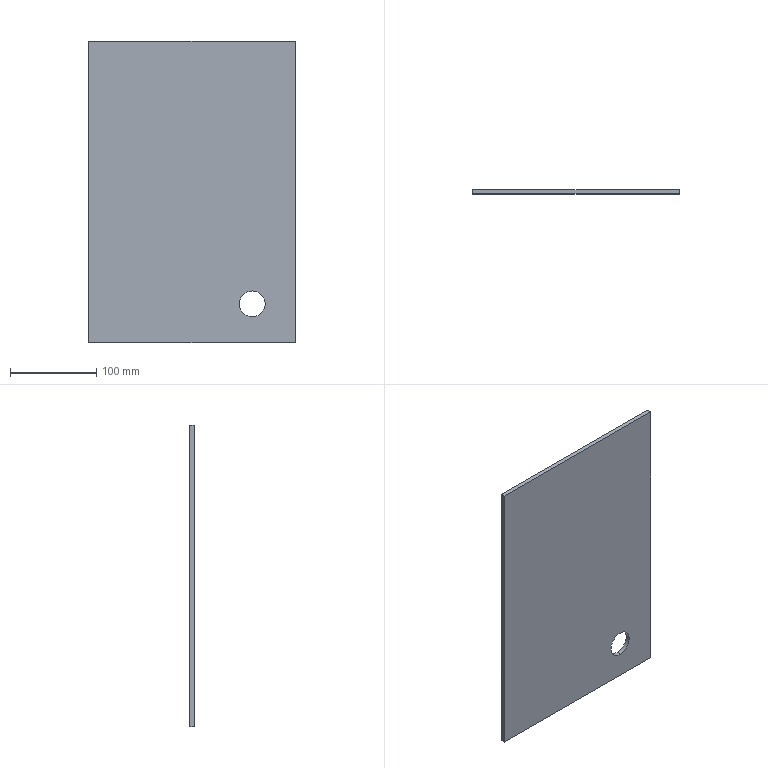Component | SolidWorks | 002FrameBaseAssembly-1_002FrameBasePanel-1 | 1 solid | 8 faces | box 240 x 5 x 350 mm | volume 416466 mm3 | plane 6 | cylinder 2 | commonest cylinder face diameters 30 x2 | material Plain Carbon Steel
build123d program:
from build123d import *

# Parameters (mm, degrees)
SKETCH1_2_W               = 400
SKETCH1_2_H               = 240
BOSS_EXTRUDE1_DEPTH       = 5
CUT_EXTRUDE2_REACH        = 235.292
SKETCH3_R                 = 15
RELIEF_GB6_WEB_DEPTH      = 234.292
RELIEF_GB6_WEB_DEPTH_BACK = 234.292
SKETCH1_W                 = 65
SKETCH1_H                 = 270


with BuildPart() as part:
    # Sketch1_2 → Boss-Extrude1 (new body)
    with BuildSketch(Plane.XY):
        Rectangle(SKETCH1_2_W, SKETCH1_2_H)
    extrude(amount=BOSS_EXTRUDE1_DEPTH)

    # Sketch3 → Cut-Extrude2 (cut, up to next)
    with BuildSketch(Plane.XY.offset(5), mode=Mode.PRIVATE) as cut_extrude2_sk1:
        with Locations((155, 70)):
            Circle(SKETCH3_R)
    cut_extrude2_tool1 = extrude(cut_extrude2_sk1.sketch, amount=-CUT_EXTRUDE2_REACH, mode=Mode.PRIVATE) & part.part
    add(cut_extrude2_tool1.solids().sort_by_distance((155, 70, 5))[0], mode=Mode.SUBTRACT)

    # Sketch1 → Relief_gb6_web (cut, two sides: drawn at the far end of the back side and taken through both)
    with BuildSketch(Plane.XY.offset(-RELIEF_GB6_WEB_DEPTH_BACK)):
        with Locations((-182.5, 0)):
            Rectangle(SKETCH1_W, SKETCH1_H)
    extrude(amount=RELIEF_GB6_WEB_DEPTH + RELIEF_GB6_WEB_DEPTH_BACK, mode=Mode.SUBTRACT)


solid = part.part

# Placed as in the assembly
solid = solid.moved(Location((0, 37, -315), (90, 0, -90)))
STEP:
#1=CARTESIAN_POINT('',(2.756,1.457,-19.094));
#2=VERTEX_POINT('',#1);
#3=CARTESIAN_POINT('',(2.756,1.457,-17.913));
#4=VERTEX_POINT('',#3);
#5=CARTESIAN_POINT('',(2.756,1.457,-18.504));
#6=DIRECTION('',(0.,1.,-0.));
#7=DIRECTION('',(0.,0.,-1.));
#8=AXIS2_PLACEMENT_3D('',#5,#6,#7);
#9=CIRCLE('',#8,0.5906);
#10=EDGE_CURVE('',#2,#4,#9,.T.);
#11=ORIENTED_EDGE('',*,*,#10,.T.);
#12=CARTESIAN_POINT('',(2.756,1.26,-17.913));
#13=VERTEX_POINT('',#12);
#14=CARTESIAN_POINT('',(2.756,1.457,-17.913));
#15=DIRECTION('',(-0.,-1.,0.));
#16=VECTOR('',#15,39.37);
#17=LINE('',#14,#16);
#18=EDGE_CURVE('',#4,#13,#17,.T.);
#19=ORIENTED_EDGE('',*,*,#18,.T.);
#20=CARTESIAN_POINT('',(2.756,1.26,-19.094));
#21=VERTEX_POINT('',#20);
#22=CARTESIAN_POINT('',(2.756,1.26,-18.504));
#23=DIRECTION('',(-0.,-1.,0.));
#24=DIRECTION('',(0.,0.,-1.));
#25=AXIS2_PLACEMENT_3D('',#22,#23,#24);
#26=CIRCLE('',#25,0.5906);
#27=EDGE_CURVE('',#13,#21,#26,.T.);
#28=ORIENTED_EDGE('',*,*,#27,.T.);
#29=CARTESIAN_POINT('',(2.756,1.457,-19.094));
#30=DIRECTION('',(-0.,-1.,0.));
#31=VECTOR('',#30,39.37);
#32=LINE('',#29,#31);
#33=EDGE_CURVE('',#2,#21,#32,.T.);
#34=ORIENTED_EDGE('',*,*,#33,.F.);
#35=EDGE_LOOP('',(#11,#19,#28,#34));
#36=FACE_OUTER_BOUND('',#35,.T.);
#37=CARTESIAN_POINT('',(2.756,1.457,-18.504));
#38=DIRECTION('',(-0.,-1.,0.));
#39=DIRECTION('',(0.,0.,-1.));
#40=AXIS2_PLACEMENT_3D('',#37,#38,#39);
#41=CYLINDRICAL_SURFACE('',#40,0.5906);
#42=ADVANCED_FACE('',(#36),#41,.F.);
#43=CARTESIAN_POINT('',(-4.724,1.457,-20.276));
#44=VERTEX_POINT('',#43);
#45=CARTESIAN_POINT('',(4.724,1.457,-20.276));
#46=VERTEX_POINT('',#45);
#47=CARTESIAN_POINT('',(4.724,1.457,-20.276));
#48=DIRECTION('',(1.,-0.,0.));
#49=VECTOR('',#48,39.37);
#50=LINE('',#47,#49);
#51=EDGE_CURVE('',#44,#46,#50,.T.);
#52=ORIENTED_EDGE('',*,*,#51,.T.);
#53=CARTESIAN_POINT('',(4.724,1.26,-20.276));
#54=VERTEX_POINT('',#53);
#55=CARTESIAN_POINT('',(4.724,1.26,-20.276));
#56=DIRECTION('',(0.,1.,-0.));
#57=VECTOR('',#56,39.37);
#58=LINE('',#55,#57);
#59=EDGE_CURVE('',#54,#46,#58,.T.);
#60=ORIENTED_EDGE('',*,*,#59,.F.);
#61=CARTESIAN_POINT('',(-4.724,1.26,-20.276));
#62=VERTEX_POINT('',#61);
#63=CARTESIAN_POINT('',(4.724,1.26,-20.276));
#64=DIRECTION('',(1.,-0.,0.));
#65=VECTOR('',#64,39.37);
#66=LINE('',#63,#65);
#67=EDGE_CURVE('',#62,#54,#66,.T.);
#68=ORIENTED_EDGE('',*,*,#67,.F.);
#69=CARTESIAN_POINT('',(-4.724,1.26,-20.276));
#70=DIRECTION('',(0.,1.,-0.));
#71=VECTOR('',#70,39.37);
#72=LINE('',#69,#71);
#73=EDGE_CURVE('',#62,#44,#72,.T.);
#74=ORIENTED_EDGE('',*,*,#73,.T.);
#75=EDGE_LOOP('',(#52,#60,#68,#74));
#76=FACE_OUTER_BOUND('',#75,.T.);
#77=CARTESIAN_POINT('',(4.724,1.26,-20.276));
#78=DIRECTION('',(0.,0.,1.));
#79=DIRECTION('',(-0.,-1.,0.));
#80=AXIS2_PLACEMENT_3D('',#77,#78,#79);
#81=PLANE('',#80);
#82=ADVANCED_FACE('',(#76),#81,.F.);
#83=CARTESIAN_POINT('',(4.724,1.457,-6.496));
#84=VERTEX_POINT('',#83);
#85=CARTESIAN_POINT('',(4.724,1.457,-4.528));
#86=DIRECTION('',(0.,0.,1.));
#87=VECTOR('',#86,39.37);
#88=LINE('',#85,#87);
#89=EDGE_CURVE('',#46,#84,#88,.T.);
#90=ORIENTED_EDGE('',*,*,#89,.T.);
#91=CARTESIAN_POINT('',(4.724,1.26,-6.496));
#92=VERTEX_POINT('',#91);
#93=CARTESIAN_POINT('',(4.724,1.26,-6.496));
#94=DIRECTION('',(-0.,-1.,0.));
#95=VECTOR('',#94,39.37);
#96=LINE('',#93,#95);
#97=EDGE_CURVE('',#84,#92,#96,.T.);
#98=ORIENTED_EDGE('',*,*,#97,.T.);
#99=CARTESIAN_POINT('',(4.724,1.26,-4.528));
#100=DIRECTION('',(0.,0.,1.));
#101=VECTOR('',#100,39.37);
#102=LINE('',#99,#101);
#103=EDGE_CURVE('',#54,#92,#102,.T.);
#104=ORIENTED_EDGE('',*,*,#103,.F.);
#105=ORIENTED_EDGE('',*,*,#59,.T.);
#106=EDGE_LOOP('',(#90,#98,#104,#105));
#107=FACE_OUTER_BOUND('',#106,.T.);
#108=CARTESIAN_POINT('',(4.724,1.26,-4.528));
#109=DIRECTION('',(-1.,0.,0.));
#110=DIRECTION('',(0.,1.,-0.));
#111=AXIS2_PLACEMENT_3D('',#108,#109,#110);
#112=PLANE('',#111);
#113=ADVANCED_FACE('',(#107),#112,.F.);
#114=CARTESIAN_POINT('',(-4.724,1.26,-6.496));
#115=VERTEX_POINT('',#114);
#116=CARTESIAN_POINT('',(-4.724,1.26,-4.528));
#117=DIRECTION('',(-0.,-0.,-1.));
#118=VECTOR('',#117,39.37);
#119=LINE('',#116,#118);
#120=EDGE_CURVE('',#115,#62,#119,.T.);
#121=ORIENTED_EDGE('',*,*,#120,.F.);
#122=CARTESIAN_POINT('',(-4.724,1.457,-6.496));
#123=VERTEX_POINT('',#122);
#124=CARTESIAN_POINT('',(-4.724,1.26,-6.496));
#125=DIRECTION('',(0.,1.,-0.));
#126=VECTOR('',#125,39.37);
#127=LINE('',#124,#126);
#128=EDGE_CURVE('',#115,#123,#127,.T.);
#129=ORIENTED_EDGE('',*,*,#128,.T.);
#130=CARTESIAN_POINT('',(-4.724,1.457,-4.528));
#131=DIRECTION('',(-0.,-0.,-1.));
#132=VECTOR('',#131,39.37);
#133=LINE('',#130,#132);
#134=EDGE_CURVE('',#123,#44,#133,.T.);
#135=ORIENTED_EDGE('',*,*,#134,.T.);
#136=ORIENTED_EDGE('',*,*,#73,.F.);
#137=EDGE_LOOP('',(#121,#129,#135,#136));
#138=FACE_OUTER_BOUND('',#137,.T.);
#139=CARTESIAN_POINT('',(-4.724,1.26,-4.528));
#140=DIRECTION('',(1.,-0.,0.));
#141=DIRECTION('',(-0.,-1.,0.));
#142=AXIS2_PLACEMENT_3D('',#139,#140,#141);
#143=PLANE('',#142);
#144=ADVANCED_FACE('',(#138),#143,.F.);
#145=CARTESIAN_POINT('',(-5.315,1.26,-6.496));
#146=DIRECTION('',(1.,-0.,0.));
#147=VECTOR('',#146,39.37);
#148=LINE('',#145,#147);
#149=EDGE_CURVE('',#115,#92,#148,.T.);
#150=ORIENTED_EDGE('',*,*,#149,.F.);
#151=ORIENTED_EDGE('',*,*,#120,.T.);
#152=ORIENTED_EDGE('',*,*,#67,.T.);
#153=ORIENTED_EDGE('',*,*,#103,.T.);
#154=EDGE_LOOP('',(#150,#151,#152,#153));
#155=FACE_OUTER_BOUND('',#154,.T.);
#156=CARTESIAN_POINT('',(2.756,1.26,-18.504));
#157=DIRECTION('',(-0.,-1.,0.));
#158=DIRECTION('',(0.,0.,-1.));
#159=AXIS2_PLACEMENT_3D('',#156,#157,#158);
#160=CIRCLE('',#159,0.5906);
#161=EDGE_CURVE('',#21,#13,#160,.T.);
#162=ORIENTED_EDGE('',*,*,#161,.F.);
#163=ORIENTED_EDGE('',*,*,#27,.F.);
#164=EDGE_LOOP('',(#162,#163));
#165=FACE_BOUND('',#164,.T.);
#166=CARTESIAN_POINT('',(-4.724,1.26,-20.276));
#167=DIRECTION('',(-0.,-1.,0.));
#168=DIRECTION('',(-0.,-0.,-1.));
#169=AXIS2_PLACEMENT_3D('',#166,#167,#168);
#170=PLANE('',#169);
#171=ADVANCED_FACE('',(#155,#165),#170,.T.);
#172=ORIENTED_EDGE('',*,*,#10,.F.);
#173=CARTESIAN_POINT('',(2.756,1.457,-18.504));
#174=DIRECTION('',(0.,1.,-0.));
#175=DIRECTION('',(0.,0.,-1.));
#176=AXIS2_PLACEMENT_3D('',#173,#174,#175);
#177=CIRCLE('',#176,0.5906);
#178=EDGE_CURVE('',#4,#2,#177,.T.);
#179=ORIENTED_EDGE('',*,*,#178,.F.);
#180=EDGE_LOOP('',(#172,#179));
#181=FACE_BOUND('',#180,.T.);
#182=ORIENTED_EDGE('',*,*,#134,.F.);
#183=CARTESIAN_POINT('',(-4.724,1.457,-6.496));
#184=DIRECTION('',(1.,-0.,0.));
#185=VECTOR('',#184,39.37);
#186=LINE('',#183,#185);
#187=EDGE_CURVE('',#123,#84,#186,.T.);
#188=ORIENTED_EDGE('',*,*,#187,.T.);
#189=ORIENTED_EDGE('',*,*,#89,.F.);
#190=ORIENTED_EDGE('',*,*,#51,.F.);
#191=EDGE_LOOP('',(#182,#188,#189,#190));
#192=FACE_OUTER_BOUND('',#191,.T.);
#193=CARTESIAN_POINT('',(-4.724,1.457,-20.276));
#194=DIRECTION('',(-0.,-1.,0.));
#195=DIRECTION('',(-0.,-0.,-1.));
#196=AXIS2_PLACEMENT_3D('',#193,#194,#195);
#197=PLANE('',#196);
#198=ADVANCED_FACE('',(#181,#192),#197,.F.);
#199=ORIENTED_EDGE('',*,*,#18,.F.);
#200=ORIENTED_EDGE('',*,*,#178,.T.);
#201=ORIENTED_EDGE('',*,*,#33,.T.);
#202=ORIENTED_EDGE('',*,*,#161,.T.);
#203=EDGE_LOOP('',(#199,#200,#201,#202));
#204=FACE_OUTER_BOUND('',#203,.T.);
#205=CARTESIAN_POINT('',(2.756,1.457,-18.504));
#206=DIRECTION('',(-0.,-1.,0.));
#207=DIRECTION('',(0.,0.,-1.));
#208=AXIS2_PLACEMENT_3D('',#205,#206,#207);
#209=CYLINDRICAL_SURFACE('',#208,0.5906);
#210=ADVANCED_FACE('',(#204),#209,.F.);
#211=ORIENTED_EDGE('',*,*,#187,.F.);
#212=ORIENTED_EDGE('',*,*,#128,.F.);
#213=ORIENTED_EDGE('',*,*,#149,.T.);
#214=ORIENTED_EDGE('',*,*,#97,.F.);
#215=EDGE_LOOP('',(#211,#212,#213,#214));
#216=FACE_OUTER_BOUND('',#215,.T.);
#217=CARTESIAN_POINT('',(-5.315,1.457,-6.496));
#218=DIRECTION('',(-0.,-0.,-1.));
#219=DIRECTION('',(0.,1.,-0.));
#220=AXIS2_PLACEMENT_3D('',#217,#218,#219);
#221=PLANE('',#220);
#222=ADVANCED_FACE('',(#216),#221,.F.);
#223=CLOSED_SHELL('',(#42,#82,#113,#144,#171,#198,#210,#222));
#224=MANIFOLD_SOLID_BREP('',#223);
#225=CARTESIAN_POINT('',(0.,0.,0.));
#226=DIRECTION('',(0.,0.,1.));
#227=DIRECTION('',(1.,0.,0.));
#228=AXIS2_PLACEMENT_3D('',#225,#226,#227);
#229=(LENGTH_UNIT()NAMED_UNIT(*)SI_UNIT($,.METRE.));
#230=LENGTH_MEASURE_WITH_UNIT(LENGTH_MEASURE(0.0254),#229);
#231=DIMENSIONAL_EXPONENTS(1.,0.,0.,0.,0.,0.,0.);
#232=(CONVERSION_BASED_UNIT('',#230)LENGTH_UNIT()NAMED_UNIT(#231));
#233=UNCERTAINTY_MEASURE_WITH_UNIT(LENGTH_MEASURE(0.00001),#232,'','');
#234=(NAMED_UNIT(*)PLANE_ANGLE_UNIT()SI_UNIT($,.RADIAN.));
#235=(NAMED_UNIT(*)SI_UNIT($,.STERADIAN.)SOLID_ANGLE_UNIT());
#236=(GEOMETRIC_REPRESENTATION_CONTEXT(3)GLOBAL_UNCERTAINTY_ASSIGNED_CONTEXT((#233))GLOBAL_UNIT_ASSIGNED_CONTEXT((#232,#234,#235))REPRESENTATION_CONTEXT('',''));
#237=ADVANCED_BREP_SHAPE_REPRESENTATION('',(#224,#228),#236);
#238=COLOUR_RGB('',0.7922,0.8196,0.9333);
#239=FILL_AREA_STYLE_COLOUR('',#238);
#240=FILL_AREA_STYLE('',(#239));
#241=SURFACE_STYLE_FILL_AREA(#240);
#242=SURFACE_SIDE_STYLE('',(#241));
#243=SURFACE_STYLE_USAGE(.BOTH.,#242);
#244=PRESENTATION_STYLE_ASSIGNMENT((#243));
#245=STYLED_ITEM('',(#244),#224);
#246=PRESENTATION_LAYER_ASSIGNMENT('','',(#245));
#247=(LENGTH_UNIT()NAMED_UNIT(*)SI_UNIT($,.METRE.));
#248=LENGTH_MEASURE_WITH_UNIT(LENGTH_MEASURE(0.0254),#247);
#249=DIMENSIONAL_EXPONENTS(1.,0.,0.,0.,0.,0.,0.);
#250=(CONVERSION_BASED_UNIT('',#248)LENGTH_UNIT()NAMED_UNIT(#249));
#251=UNCERTAINTY_MEASURE_WITH_UNIT(LENGTH_MEASURE(0.00001),#250,'','');
#252=(NAMED_UNIT(*)PLANE_ANGLE_UNIT()SI_UNIT($,.RADIAN.));
#253=(NAMED_UNIT(*)SI_UNIT($,.STERADIAN.)SOLID_ANGLE_UNIT());
#254=(GEOMETRIC_REPRESENTATION_CONTEXT(3)GLOBAL_UNCERTAINTY_ASSIGNED_CONTEXT((#251))GLOBAL_UNIT_ASSIGNED_CONTEXT((#250,#252,#253))REPRESENTATION_CONTEXT('',''));
#255=MECHANICAL_DESIGN_GEOMETRIC_PRESENTATION_REPRESENTATION('',(#245),#254);